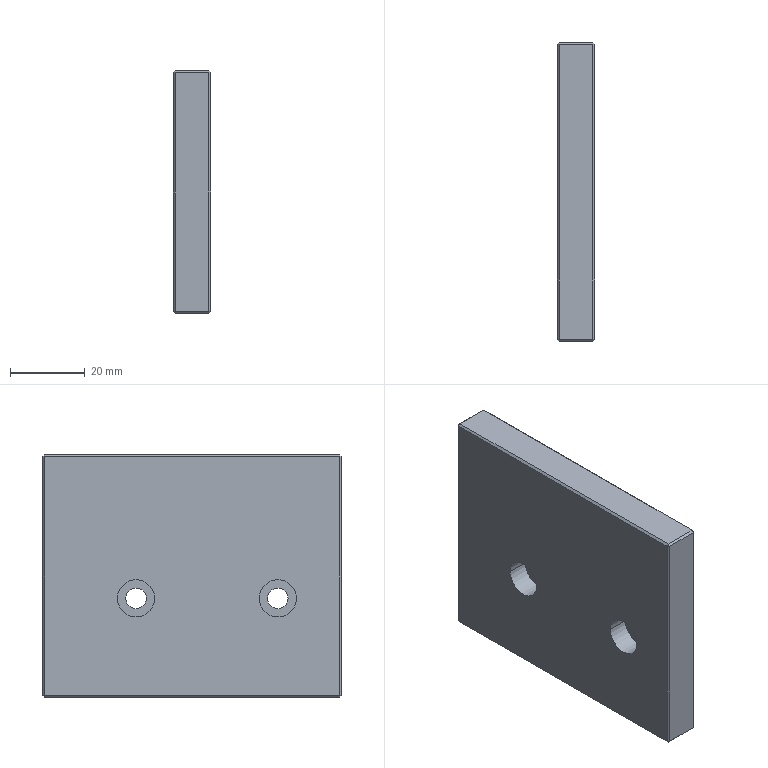Component | SolidWorks | BearingHousingAssembly-1_AirGripperFixingPlate2-1 | 1 solid | 62 faces | box 10 x 80 x 65 mm | volume 49667 mm3 | plane 28 | cylinder 18 | cone 16 | commonest cylinder face diameters 4.2 x10 10 x4 5.5 x4 | material 1060 Alloy
build123d program:
from build123d import *

# Parameters (mm, degrees)
SKETCH1_W                                          = 80
SKETCH1_H                                          = 65
BOSS_EXTRUDE1_DEPTH                                = 5
M5_TAPPED_HOLE1_D                                  = 4.2
M5_TAPPED_HOLE1_DEPTH                              = 17.4
M5_TAPPED_HOLE1_TIP                                = 1.262
CHAMFER1_SIZE                                      = 0.5
M4_TAPPED_HOLE1_D                                  = 3.3
M5_TAPPED_HOLE2_D                                  = 4.2
M5_TAPPED_HOLE2_DEPTH                              = 14.4
M5_TAPPED_HOLE2_TIP                                = 1.262
HOLE_SIZE_ACCORDING_TO_TYPE_OF_HEXAGON_D           = 5.5
HOLE_SIZE_ACCORDING_TO_TYPE_OF_HEXAGON_CBORE_D     = 10
HOLE_SIZE_ACCORDING_TO_TYPE_OF_HEXAGON_CBORE_DEPTH = 5.7


with BuildPart() as part:
    # Sketch1 → Boss-Extrude1 (new, symmetric)
    with BuildSketch(Plane.XY):
        with Locations((40, 7.5)):
            Rectangle(SKETCH1_W, SKETCH1_H)
    extrude(amount=BOSS_EXTRUDE1_DEPTH, both=True)

    # M5 Tapped Hole1
    with Locations(Plane.ZY):
        with Locations((0, 17.5), (0, 0), (0, -17.5)):
            Hole(M5_TAPPED_HOLE1_D / 2, depth=M5_TAPPED_HOLE1_DEPTH)
            with Locations((0, 0, -(M5_TAPPED_HOLE1_DEPTH + M5_TAPPED_HOLE1_TIP / 2))):  # 118° drill point
                Cone(0, M5_TAPPED_HOLE1_D / 2, M5_TAPPED_HOLE1_TIP, mode=Mode.SUBTRACT)

    # Chamfer1
    chamfer1_edges = [part.edges().sort_by_distance(p)[0] for p in [
        (80, 7.5, 5),
        (40, 40, 5),
        (0, -17.5, 2.1),
        (0, 0, 2.1),
        (0, 17.5, 2.1),
        (0, 7.5, 5),
        (40, 40, -5),
        (80, 7.5, -5),
        (40, -25, -5),
        (0, 7.5, -5),
        (40, -25, 5),
        (0, 40, 0),
        (80, 40, 0),
        (80, -25, 0),
        (0, -25, 0),
    ]]
    chamfer(chamfer1_edges, length=CHAMFER1_SIZE)

    # M4 Tapped Hole1 (through all)
    with Locations(Plane(origin=(0, 0, -5), x_dir=(-1, 0, 0), z_dir=(0, 0, -1))):
        with Locations((-25, 13.5), (-63, 13.5)):
            Hole(M4_TAPPED_HOLE1_D / 2)

    # M5 Tapped Hole2
    with Locations(Plane(origin=(0, 40, 0), x_dir=(1, 0, 0), z_dir=(0, 1, 0))):
        with Locations((70, 0), (30, 0)):
            Hole(M5_TAPPED_HOLE2_D / 2, depth=M5_TAPPED_HOLE2_DEPTH)
            with Locations((0, 0, -(M5_TAPPED_HOLE2_DEPTH + M5_TAPPED_HOLE2_TIP / 2))):  # 118° drill point
                Cone(0, M5_TAPPED_HOLE2_D / 2, M5_TAPPED_HOLE2_TIP, mode=Mode.SUBTRACT)

    # Hole Size _according to_ type of Hexagon (through all)
    with Locations(Plane(origin=(0, 0, -5), x_dir=(-1, 0, 0), z_dir=(0, 0, -1))):
        with Locations((-63, 13.5), (-25, 13.5)):
            CounterBoreHole(HOLE_SIZE_ACCORDING_TO_TYPE_OF_HEXAGON_D / 2, HOLE_SIZE_ACCORDING_TO_TYPE_OF_HEXAGON_CBORE_D / 2, HOLE_SIZE_ACCORDING_TO_TYPE_OF_HEXAGON_CBORE_DEPTH)


solid = part.part

# Placed as in the assembly
solid = solid.moved(Location((-81.666, 121.264, -6), (-90, 90, 0)))